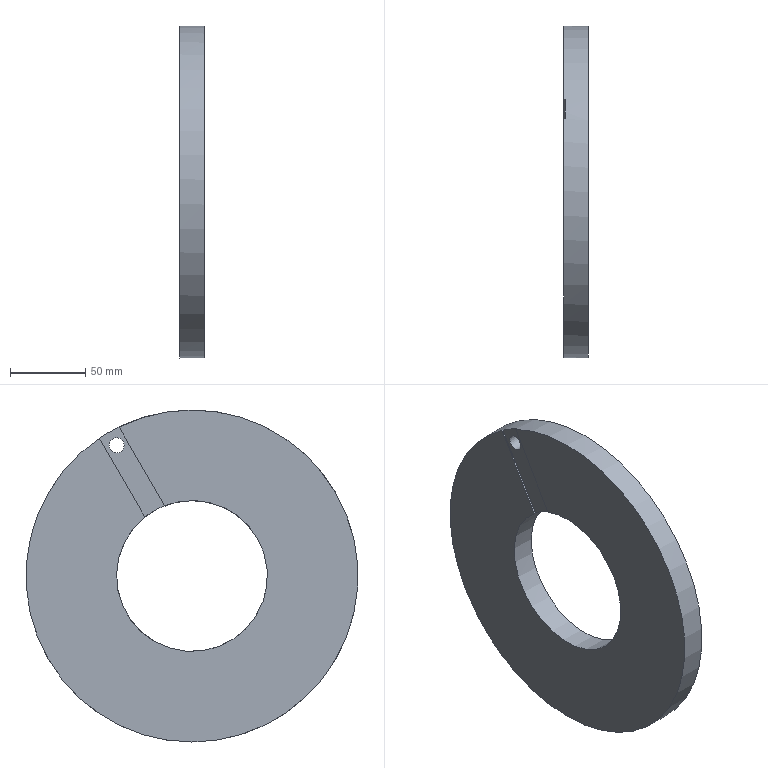Component | NX | SIM15_C3_AXIS | 1 solid | 8 faces | volume 480469 mm3 | plane 5 | cylinder 3 | commonest cylinder face diameters 220 x1 100 x1 10 x1